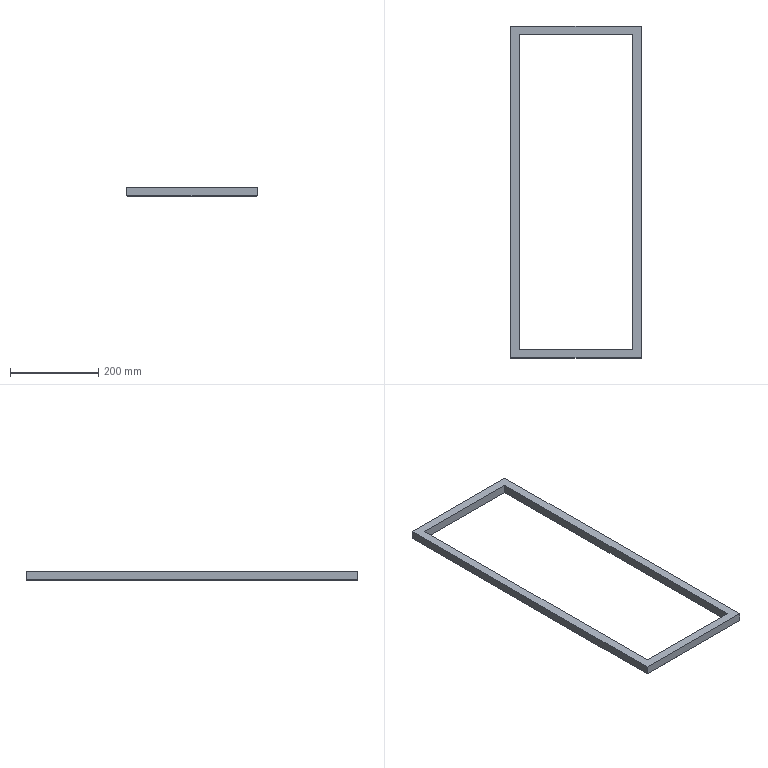Component | SolidWorks | Light-1_OuterFrame-1 | 1 solid | 14 faces | box 297 x 754 x 20 mm | volume 807750 mm3 | plane 14
STEP:
#1=COLOUR_RGB('',0.7922,0.8196,0.9333);
#2=FILL_AREA_STYLE_COLOUR('',#1);
#3=FILL_AREA_STYLE('',(#2));
#4=SURFACE_STYLE_FILL_AREA(#3);
#5=SURFACE_SIDE_STYLE('',(#4));
#6=SURFACE_STYLE_USAGE(.BOTH.,#5);
#7=PRESENTATION_STYLE_ASSIGNMENT((#6));
#8=CARTESIAN_POINT('',(-207.4,261.615,5.614));
#9=VERTEX_POINT('',#8);
#10=CARTESIAN_POINT('',(-217.518,261.615,5.614));
#11=VERTEX_POINT('',#10);
#12=CARTESIAN_POINT('',(-212.459,261.615,5.614));
#13=DIRECTION('',(-1.,0.,0.));
#14=VECTOR('',#13,39.37);
#15=LINE('',#12,#14);
#16=EDGE_CURVE('',#9,#11,#15,.T.);
#17=ORIENTED_EDGE('',*,*,#16,.T.);
#18=CARTESIAN_POINT('',(-217.518,289.725,5.614));
#19=VERTEX_POINT('',#18);
#20=CARTESIAN_POINT('',(-217.518,275.67,5.614));
#21=DIRECTION('',(0.,1.,-0.));
#22=VECTOR('',#21,39.37);
#23=LINE('',#20,#22);
#24=EDGE_CURVE('',#11,#19,#23,.T.);
#25=ORIENTED_EDGE('',*,*,#24,.T.);
#26=CARTESIAN_POINT('',(-207.4,289.725,5.614));
#27=VERTEX_POINT('',#26);
#28=CARTESIAN_POINT('',(-212.459,289.725,5.614));
#29=DIRECTION('',(1.,-0.,-0.));
#30=VECTOR('',#29,39.37);
#31=LINE('',#28,#30);
#32=EDGE_CURVE('',#19,#27,#31,.T.);
#33=ORIENTED_EDGE('',*,*,#32,.T.);
#34=CARTESIAN_POINT('',(-207.4,275.67,5.614));
#35=DIRECTION('',(-0.,-1.,0.));
#36=VECTOR('',#35,39.37);
#37=LINE('',#34,#36);
#38=EDGE_CURVE('',#27,#9,#37,.T.);
#39=ORIENTED_EDGE('',*,*,#38,.T.);
#40=EDGE_LOOP('',(#17,#25,#33,#39));
#41=FACE_BOUND('',#40,.T.);
#42=CARTESIAN_POINT('',(-218.305,260.828,5.614));
#43=VERTEX_POINT('',#42);
#44=CARTESIAN_POINT('',(-206.612,260.828,5.614));
#45=VERTEX_POINT('',#44);
#46=CARTESIAN_POINT('',(-212.459,260.828,5.614));
#47=DIRECTION('',(1.,-0.,-0.));
#48=VECTOR('',#47,39.37);
#49=LINE('',#46,#48);
#50=EDGE_CURVE('',#43,#45,#49,.T.);
#51=ORIENTED_EDGE('',*,*,#50,.T.);
#52=CARTESIAN_POINT('',(-206.612,290.513,5.614));
#53=VERTEX_POINT('',#52);
#54=CARTESIAN_POINT('',(-206.612,275.67,5.614));
#55=DIRECTION('',(0.,1.,-0.));
#56=VECTOR('',#55,39.37);
#57=LINE('',#54,#56);
#58=EDGE_CURVE('',#45,#53,#57,.T.);
#59=ORIENTED_EDGE('',*,*,#58,.T.);
#60=CARTESIAN_POINT('',(-218.305,290.513,5.614));
#61=VERTEX_POINT('',#60);
#62=CARTESIAN_POINT('',(-212.459,290.513,5.614));
#63=DIRECTION('',(-1.,0.,0.));
#64=VECTOR('',#63,39.37);
#65=LINE('',#62,#64);
#66=EDGE_CURVE('',#53,#61,#65,.T.);
#67=ORIENTED_EDGE('',*,*,#66,.T.);
#68=CARTESIAN_POINT('',(-218.305,275.67,5.614));
#69=DIRECTION('',(-0.,-1.,0.));
#70=VECTOR('',#69,39.37);
#71=LINE('',#68,#70);
#72=EDGE_CURVE('',#61,#43,#71,.T.);
#73=ORIENTED_EDGE('',*,*,#72,.T.);
#74=EDGE_LOOP('',(#51,#59,#67,#73));
#75=FACE_OUTER_BOUND('',#74,.T.);
#76=CARTESIAN_POINT('',(-218.305,290.513,5.614));
#77=DIRECTION('',(0.,0.,1.));
#78=DIRECTION('',(-0.,-1.,0.));
#79=AXIS2_PLACEMENT_3D('',#76,#77,#78);
#80=PLANE('',#79);
#81=ADVANCED_FACE('',(#41,#75),#80,.T.);
#82=ORIENTED_EDGE('',*,*,#24,.F.);
#83=CARTESIAN_POINT('',(-217.518,261.615,4.826));
#84=VERTEX_POINT('',#83);
#85=CARTESIAN_POINT('',(-217.518,261.615,5.22));
#86=DIRECTION('',(-0.,-0.,-1.));
#87=VECTOR('',#86,39.37);
#88=LINE('',#85,#87);
#89=EDGE_CURVE('',#11,#84,#88,.T.);
#90=ORIENTED_EDGE('',*,*,#89,.T.);
#91=CARTESIAN_POINT('',(-217.518,289.725,4.826));
#92=VERTEX_POINT('',#91);
#93=CARTESIAN_POINT('',(-217.518,275.67,4.826));
#94=DIRECTION('',(0.,1.,-0.));
#95=VECTOR('',#94,39.37);
#96=LINE('',#93,#95);
#97=EDGE_CURVE('',#84,#92,#96,.T.);
#98=ORIENTED_EDGE('',*,*,#97,.T.);
#99=CARTESIAN_POINT('',(-217.518,289.725,5.22));
#100=DIRECTION('',(0.,0.,1.));
#101=VECTOR('',#100,39.37);
#102=LINE('',#99,#101);
#103=EDGE_CURVE('',#92,#19,#102,.T.);
#104=ORIENTED_EDGE('',*,*,#103,.T.);
#105=EDGE_LOOP('',(#82,#90,#98,#104));
#106=FACE_OUTER_BOUND('',#105,.T.);
#107=CARTESIAN_POINT('',(-217.518,289.725,4.826));
#108=DIRECTION('',(1.,-0.,-0.));
#109=DIRECTION('',(0.,0.,1.));
#110=AXIS2_PLACEMENT_3D('',#107,#108,#109);
#111=PLANE('',#110);
#112=ADVANCED_FACE('',(#106),#111,.T.);
#113=ORIENTED_EDGE('',*,*,#16,.F.);
#114=CARTESIAN_POINT('',(-207.4,261.615,4.826));
#115=VERTEX_POINT('',#114);
#116=CARTESIAN_POINT('',(-207.4,261.615,5.22));
#117=DIRECTION('',(-0.,-0.,-1.));
#118=VECTOR('',#117,39.37);
#119=LINE('',#116,#118);
#120=EDGE_CURVE('',#9,#115,#119,.T.);
#121=ORIENTED_EDGE('',*,*,#120,.T.);
#122=CARTESIAN_POINT('',(-212.459,261.615,4.826));
#123=DIRECTION('',(-1.,0.,0.));
#124=VECTOR('',#123,39.37);
#125=LINE('',#122,#124);
#126=EDGE_CURVE('',#115,#84,#125,.T.);
#127=ORIENTED_EDGE('',*,*,#126,.T.);
#128=ORIENTED_EDGE('',*,*,#89,.F.);
#129=EDGE_LOOP('',(#113,#121,#127,#128));
#130=FACE_OUTER_BOUND('',#129,.T.);
#131=CARTESIAN_POINT('',(-217.518,261.615,4.826));
#132=DIRECTION('',(0.,1.,-0.));
#133=DIRECTION('',(0.,0.,1.));
#134=AXIS2_PLACEMENT_3D('',#131,#132,#133);
#135=PLANE('',#134);
#136=ADVANCED_FACE('',(#130),#135,.T.);
#137=ORIENTED_EDGE('',*,*,#38,.F.);
#138=CARTESIAN_POINT('',(-207.4,289.725,4.826));
#139=VERTEX_POINT('',#138);
#140=CARTESIAN_POINT('',(-207.4,289.725,5.22));
#141=DIRECTION('',(-0.,-0.,-1.));
#142=VECTOR('',#141,39.37);
#143=LINE('',#140,#142);
#144=EDGE_CURVE('',#27,#139,#143,.T.);
#145=ORIENTED_EDGE('',*,*,#144,.T.);
#146=CARTESIAN_POINT('',(-207.4,275.67,4.826));
#147=DIRECTION('',(-0.,-1.,0.));
#148=VECTOR('',#147,39.37);
#149=LINE('',#146,#148);
#150=EDGE_CURVE('',#139,#115,#149,.T.);
#151=ORIENTED_EDGE('',*,*,#150,.T.);
#152=ORIENTED_EDGE('',*,*,#120,.F.);
#153=EDGE_LOOP('',(#137,#145,#151,#152));
#154=FACE_OUTER_BOUND('',#153,.T.);
#155=CARTESIAN_POINT('',(-207.4,289.725,5.614));
#156=DIRECTION('',(-1.,0.,0.));
#157=DIRECTION('',(-0.,-0.,-1.));
#158=AXIS2_PLACEMENT_3D('',#155,#156,#157);
#159=PLANE('',#158);
#160=ADVANCED_FACE('',(#154),#159,.T.);
#161=ORIENTED_EDGE('',*,*,#32,.F.);
#162=ORIENTED_EDGE('',*,*,#103,.F.);
#163=CARTESIAN_POINT('',(-212.459,289.725,4.826));
#164=DIRECTION('',(1.,-0.,-0.));
#165=VECTOR('',#164,39.37);
#166=LINE('',#163,#165);
#167=EDGE_CURVE('',#92,#139,#166,.T.);
#168=ORIENTED_EDGE('',*,*,#167,.T.);
#169=ORIENTED_EDGE('',*,*,#144,.F.);
#170=EDGE_LOOP('',(#161,#162,#168,#169));
#171=FACE_OUTER_BOUND('',#170,.T.);
#172=CARTESIAN_POINT('',(-217.518,289.725,5.614));
#173=DIRECTION('',(-0.,-1.,0.));
#174=DIRECTION('',(-0.,-0.,-1.));
#175=AXIS2_PLACEMENT_3D('',#172,#173,#174);
#176=PLANE('',#175);
#177=ADVANCED_FACE('',(#171),#176,.T.);
#178=CARTESIAN_POINT('',(-206.612,260.828,4.866));
#179=VERTEX_POINT('',#178);
#180=CARTESIAN_POINT('',(-206.612,260.828,5.22));
#181=DIRECTION('',(0.,0.,1.));
#182=VECTOR('',#181,39.37);
#183=LINE('',#180,#182);
#184=EDGE_CURVE('',#179,#45,#183,.T.);
#185=ORIENTED_EDGE('',*,*,#184,.F.);
#186=CARTESIAN_POINT('',(-206.612,290.513,4.866));
#187=VERTEX_POINT('',#186);
#188=CARTESIAN_POINT('',(-206.612,290.513,4.866));
#189=DIRECTION('',(0.,1.,-0.));
#190=VECTOR('',#189,39.37);
#191=LINE('',#188,#190);
#192=EDGE_CURVE('',#179,#187,#191,.T.);
#193=ORIENTED_EDGE('',*,*,#192,.T.);
#194=CARTESIAN_POINT('',(-206.612,290.513,5.22));
#195=DIRECTION('',(-0.,-0.,-1.));
#196=VECTOR('',#195,39.37);
#197=LINE('',#194,#196);
#198=EDGE_CURVE('',#53,#187,#197,.T.);
#199=ORIENTED_EDGE('',*,*,#198,.F.);
#200=ORIENTED_EDGE('',*,*,#58,.F.);
#201=EDGE_LOOP('',(#185,#193,#199,#200));
#202=FACE_OUTER_BOUND('',#201,.T.);
#203=CARTESIAN_POINT('',(-206.612,290.513,4.826));
#204=DIRECTION('',(-1.,0.,0.));
#205=DIRECTION('',(-0.,-1.,0.));
#206=AXIS2_PLACEMENT_3D('',#203,#204,#205);
#207=PLANE('',#206);
#208=ADVANCED_FACE('',(#202),#207,.F.);
#209=CARTESIAN_POINT('',(-218.305,260.828,4.866));
#210=VERTEX_POINT('',#209);
#211=CARTESIAN_POINT('',(-218.305,260.828,5.22));
#212=DIRECTION('',(0.,0.,1.));
#213=VECTOR('',#212,39.37);
#214=LINE('',#211,#213);
#215=EDGE_CURVE('',#210,#43,#214,.T.);
#216=ORIENTED_EDGE('',*,*,#215,.F.);
#217=CARTESIAN_POINT('',(-206.612,260.828,4.866));
#218=DIRECTION('',(1.,-0.,-0.));
#219=VECTOR('',#218,39.37);
#220=LINE('',#217,#219);
#221=EDGE_CURVE('',#210,#179,#220,.T.);
#222=ORIENTED_EDGE('',*,*,#221,.T.);
#223=ORIENTED_EDGE('',*,*,#184,.T.);
#224=ORIENTED_EDGE('',*,*,#50,.F.);
#225=EDGE_LOOP('',(#216,#222,#223,#224));
#226=FACE_OUTER_BOUND('',#225,.T.);
#227=CARTESIAN_POINT('',(-206.612,260.828,4.826));
#228=DIRECTION('',(0.,1.,-0.));
#229=DIRECTION('',(-1.,0.,0.));
#230=AXIS2_PLACEMENT_3D('',#227,#228,#229);
#231=PLANE('',#230);
#232=ADVANCED_FACE('',(#226),#231,.F.);
#233=CARTESIAN_POINT('',(-218.305,290.513,4.866));
#234=VERTEX_POINT('',#233);
#235=CARTESIAN_POINT('',(-218.305,290.513,5.22));
#236=DIRECTION('',(0.,0.,1.));
#237=VECTOR('',#236,39.37);
#238=LINE('',#235,#237);
#239=EDGE_CURVE('',#234,#61,#238,.T.);
#240=ORIENTED_EDGE('',*,*,#239,.F.);
#241=CARTESIAN_POINT('',(-218.305,260.828,4.866));
#242=DIRECTION('',(-0.,-1.,0.));
#243=VECTOR('',#242,39.37);
#244=LINE('',#241,#243);
#245=EDGE_CURVE('',#234,#210,#244,.T.);
#246=ORIENTED_EDGE('',*,*,#245,.T.);
#247=ORIENTED_EDGE('',*,*,#215,.T.);
#248=ORIENTED_EDGE('',*,*,#72,.F.);
#249=EDGE_LOOP('',(#240,#246,#247,#248));
#250=FACE_OUTER_BOUND('',#249,.T.);
#251=CARTESIAN_POINT('',(-218.305,260.828,4.826));
#252=DIRECTION('',(1.,-0.,-0.));
#253=DIRECTION('',(0.,1.,-0.));
#254=AXIS2_PLACEMENT_3D('',#251,#252,#253);
#255=PLANE('',#254);
#256=ADVANCED_FACE('',(#250),#255,.F.);
#257=ORIENTED_EDGE('',*,*,#198,.T.);
#258=CARTESIAN_POINT('',(-218.305,290.513,4.866));
#259=DIRECTION('',(-1.,0.,0.));
#260=VECTOR('',#259,39.37);
#261=LINE('',#258,#260);
#262=EDGE_CURVE('',#187,#234,#261,.T.);
#263=ORIENTED_EDGE('',*,*,#262,.T.);
#264=ORIENTED_EDGE('',*,*,#239,.T.);
#265=ORIENTED_EDGE('',*,*,#66,.F.);
#266=EDGE_LOOP('',(#257,#263,#264,#265));
#267=FACE_OUTER_BOUND('',#266,.T.);
#268=CARTESIAN_POINT('',(-218.305,290.513,4.826));
#269=DIRECTION('',(-0.,-1.,0.));
#270=DIRECTION('',(1.,-0.,-0.));
#271=AXIS2_PLACEMENT_3D('',#268,#269,#270);
#272=PLANE('',#271);
#273=ADVANCED_FACE('',(#267),#272,.F.);
#274=CARTESIAN_POINT('',(-218.266,260.867,4.826));
#275=VERTEX_POINT('',#274);
#276=CARTESIAN_POINT('',(-218.266,290.473,4.826));
#277=VERTEX_POINT('',#276);
#278=CARTESIAN_POINT('',(-218.266,290.513,4.826));
#279=DIRECTION('',(0.,1.,-0.));
#280=VECTOR('',#279,39.37);
#281=LINE('',#278,#280);
#282=EDGE_CURVE('',#275,#277,#281,.T.);
#283=ORIENTED_EDGE('',*,*,#282,.T.);
#284=CARTESIAN_POINT('',(-206.652,290.473,4.826));
#285=VERTEX_POINT('',#284);
#286=CARTESIAN_POINT('',(-218.305,290.473,4.826));
#287=DIRECTION('',(1.,-0.,-0.));
#288=VECTOR('',#287,39.37);
#289=LINE('',#286,#288);
#290=EDGE_CURVE('',#277,#285,#289,.T.);
#291=ORIENTED_EDGE('',*,*,#290,.T.);
#292=CARTESIAN_POINT('',(-206.652,260.867,4.826));
#293=VERTEX_POINT('',#292);
#294=CARTESIAN_POINT('',(-206.652,290.513,4.826));
#295=DIRECTION('',(-0.,-1.,0.));
#296=VECTOR('',#295,39.37);
#297=LINE('',#294,#296);
#298=EDGE_CURVE('',#285,#293,#297,.T.);
#299=ORIENTED_EDGE('',*,*,#298,.T.);
#300=CARTESIAN_POINT('',(-218.305,260.867,4.826));
#301=DIRECTION('',(-1.,0.,0.));
#302=VECTOR('',#301,39.37);
#303=LINE('',#300,#302);
#304=EDGE_CURVE('',#293,#275,#303,.T.);
#305=ORIENTED_EDGE('',*,*,#304,.T.);
#306=EDGE_LOOP('',(#283,#291,#299,#305));
#307=FACE_OUTER_BOUND('',#306,.T.);
#308=ORIENTED_EDGE('',*,*,#167,.F.);
#309=ORIENTED_EDGE('',*,*,#97,.F.);
#310=ORIENTED_EDGE('',*,*,#126,.F.);
#311=ORIENTED_EDGE('',*,*,#150,.F.);
#312=EDGE_LOOP('',(#308,#309,#310,#311));
#313=FACE_BOUND('',#312,.T.);
#314=CARTESIAN_POINT('',(-218.305,290.513,4.826));
#315=DIRECTION('',(0.,0.,1.));
#316=DIRECTION('',(-0.,-1.,0.));
#317=AXIS2_PLACEMENT_3D('',#314,#315,#316);
#318=PLANE('',#317);
#319=ADVANCED_FACE('',(#307,#313),#318,.F.);
#320=CARTESIAN_POINT('',(-216.534,270.749,-5.055));
#321=DIRECTION('',(-0.5774,0.5774,-0.5774));
#322=VECTOR('',#321,39.37);
#323=LINE('',#320,#322);
#324=EDGE_CURVE('',#179,#293,#323,.T.);
#325=ORIENTED_EDGE('',*,*,#324,.F.);
#326=ORIENTED_EDGE('',*,*,#221,.F.);
#327=CARTESIAN_POINT('',(-218.279,260.854,4.84));
#328=DIRECTION('',(-0.5774,-0.5774,0.5774));
#329=VECTOR('',#328,39.37);
#330=LINE('',#327,#329);
#331=EDGE_CURVE('',#275,#210,#330,.T.);
#332=ORIENTED_EDGE('',*,*,#331,.F.);
#333=ORIENTED_EDGE('',*,*,#304,.F.);
#334=EDGE_LOOP('',(#325,#326,#332,#333));
#335=FACE_OUTER_BOUND('',#334,.T.);
#336=CARTESIAN_POINT('',(-218.305,260.867,4.826));
#337=DIRECTION('',(0.,0.7071,0.7071));
#338=DIRECTION('',(-1.,0.,0.));
#339=AXIS2_PLACEMENT_3D('',#336,#337,#338);
#340=PLANE('',#339);
#341=ADVANCED_FACE('',(#335),#340,.F.);
#342=ORIENTED_EDGE('',*,*,#331,.T.);
#343=ORIENTED_EDGE('',*,*,#245,.F.);
#344=CARTESIAN_POINT('',(-218.279,290.487,4.84));
#345=DIRECTION('',(-0.5774,0.5774,0.5774));
#346=VECTOR('',#345,39.37);
#347=LINE('',#344,#346);
#348=EDGE_CURVE('',#277,#234,#347,.T.);
#349=ORIENTED_EDGE('',*,*,#348,.F.);
#350=ORIENTED_EDGE('',*,*,#282,.F.);
#351=EDGE_LOOP('',(#342,#343,#349,#350));
#352=FACE_OUTER_BOUND('',#351,.T.);
#353=CARTESIAN_POINT('',(-218.266,290.513,4.826));
#354=DIRECTION('',(0.7071,0.,0.7071));
#355=DIRECTION('',(0.,1.,-0.));
#356=AXIS2_PLACEMENT_3D('',#353,#354,#355);
#357=PLANE('',#356);
#358=ADVANCED_FACE('',(#352),#357,.F.);
#359=ORIENTED_EDGE('',*,*,#324,.T.);
#360=ORIENTED_EDGE('',*,*,#298,.F.);
#361=CARTESIAN_POINT('',(-206.639,290.487,4.84));
#362=DIRECTION('',(-0.5774,-0.5774,-0.5774));
#363=VECTOR('',#362,39.37);
#364=LINE('',#361,#363);
#365=EDGE_CURVE('',#187,#285,#364,.T.);
#366=ORIENTED_EDGE('',*,*,#365,.F.);
#367=ORIENTED_EDGE('',*,*,#192,.F.);
#368=EDGE_LOOP('',(#359,#360,#366,#367));
#369=FACE_OUTER_BOUND('',#368,.T.);
#370=CARTESIAN_POINT('',(-206.652,290.513,4.826));
#371=DIRECTION('',(-0.7071,0.,0.7071));
#372=DIRECTION('',(-0.,-1.,0.));
#373=AXIS2_PLACEMENT_3D('',#370,#371,#372);
#374=PLANE('',#373);
#375=ADVANCED_FACE('',(#369),#374,.F.);
#376=ORIENTED_EDGE('',*,*,#348,.T.);
#377=ORIENTED_EDGE('',*,*,#262,.F.);
#378=ORIENTED_EDGE('',*,*,#365,.T.);
#379=ORIENTED_EDGE('',*,*,#290,.F.);
#380=EDGE_LOOP('',(#376,#377,#378,#379));
#381=FACE_OUTER_BOUND('',#380,.T.);
#382=CARTESIAN_POINT('',(-218.305,290.473,4.826));
#383=DIRECTION('',(-0.,-0.7071,0.7071));
#384=DIRECTION('',(1.,-0.,-0.));
#385=AXIS2_PLACEMENT_3D('',#382,#383,#384);
#386=PLANE('',#385);
#387=ADVANCED_FACE('',(#381),#386,.F.);
#388=CLOSED_SHELL('',(#81,#112,#136,#160,#177,#208,#232,#256,#273,#319,#341,#358,#375,#387));
#389=MANIFOLD_SOLID_BREP('',#388);
#390=STYLED_ITEM('',(#7),#389);
#391=(LENGTH_UNIT()NAMED_UNIT(*)SI_UNIT($,.METRE.));
#392=LENGTH_MEASURE_WITH_UNIT(LENGTH_MEASURE(0.0254),#391);
#393=DIMENSIONAL_EXPONENTS(1.,0.,0.,0.,0.,0.,0.);
#394=(CONVERSION_BASED_UNIT('',#392)LENGTH_UNIT()NAMED_UNIT(#393));
#395=UNCERTAINTY_MEASURE_WITH_UNIT(LENGTH_MEASURE(0.00001),#394,'','');
#396=(NAMED_UNIT(*)PLANE_ANGLE_UNIT()SI_UNIT($,.RADIAN.));
#397=(NAMED_UNIT(*)SI_UNIT($,.STERADIAN.)SOLID_ANGLE_UNIT());
#398=(GEOMETRIC_REPRESENTATION_CONTEXT(3)GLOBAL_UNCERTAINTY_ASSIGNED_CONTEXT((#395))GLOBAL_UNIT_ASSIGNED_CONTEXT((#394,#396,#397))REPRESENTATION_CONTEXT('',''));
#399=MECHANICAL_DESIGN_GEOMETRIC_PRESENTATION_REPRESENTATION('',(#390),#398);
#400=PRESENTATION_LAYER_ASSIGNMENT('','',(#390));
#401=CARTESIAN_POINT('',(0.,0.,0.));
#402=DIRECTION('',(0.,0.,1.));
#403=DIRECTION('',(1.,0.,0.));
#404=AXIS2_PLACEMENT_3D('',#401,#402,#403);
#405=(LENGTH_UNIT()NAMED_UNIT(*)SI_UNIT($,.METRE.));
#406=LENGTH_MEASURE_WITH_UNIT(LENGTH_MEASURE(0.0254),#405);
#407=DIMENSIONAL_EXPONENTS(1.,0.,0.,0.,0.,0.,0.);
#408=(CONVERSION_BASED_UNIT('',#406)LENGTH_UNIT()NAMED_UNIT(#407));
#409=UNCERTAINTY_MEASURE_WITH_UNIT(LENGTH_MEASURE(0.00001),#408,'','');
#410=(NAMED_UNIT(*)PLANE_ANGLE_UNIT()SI_UNIT($,.RADIAN.));
#411=(NAMED_UNIT(*)SI_UNIT($,.STERADIAN.)SOLID_ANGLE_UNIT());
#412=(GEOMETRIC_REPRESENTATION_CONTEXT(3)GLOBAL_UNCERTAINTY_ASSIGNED_CONTEXT((#409))GLOBAL_UNIT_ASSIGNED_CONTEXT((#408,#410,#411))REPRESENTATION_CONTEXT('',''));
#413=ADVANCED_BREP_SHAPE_REPRESENTATION('',(#389,#404),#412);